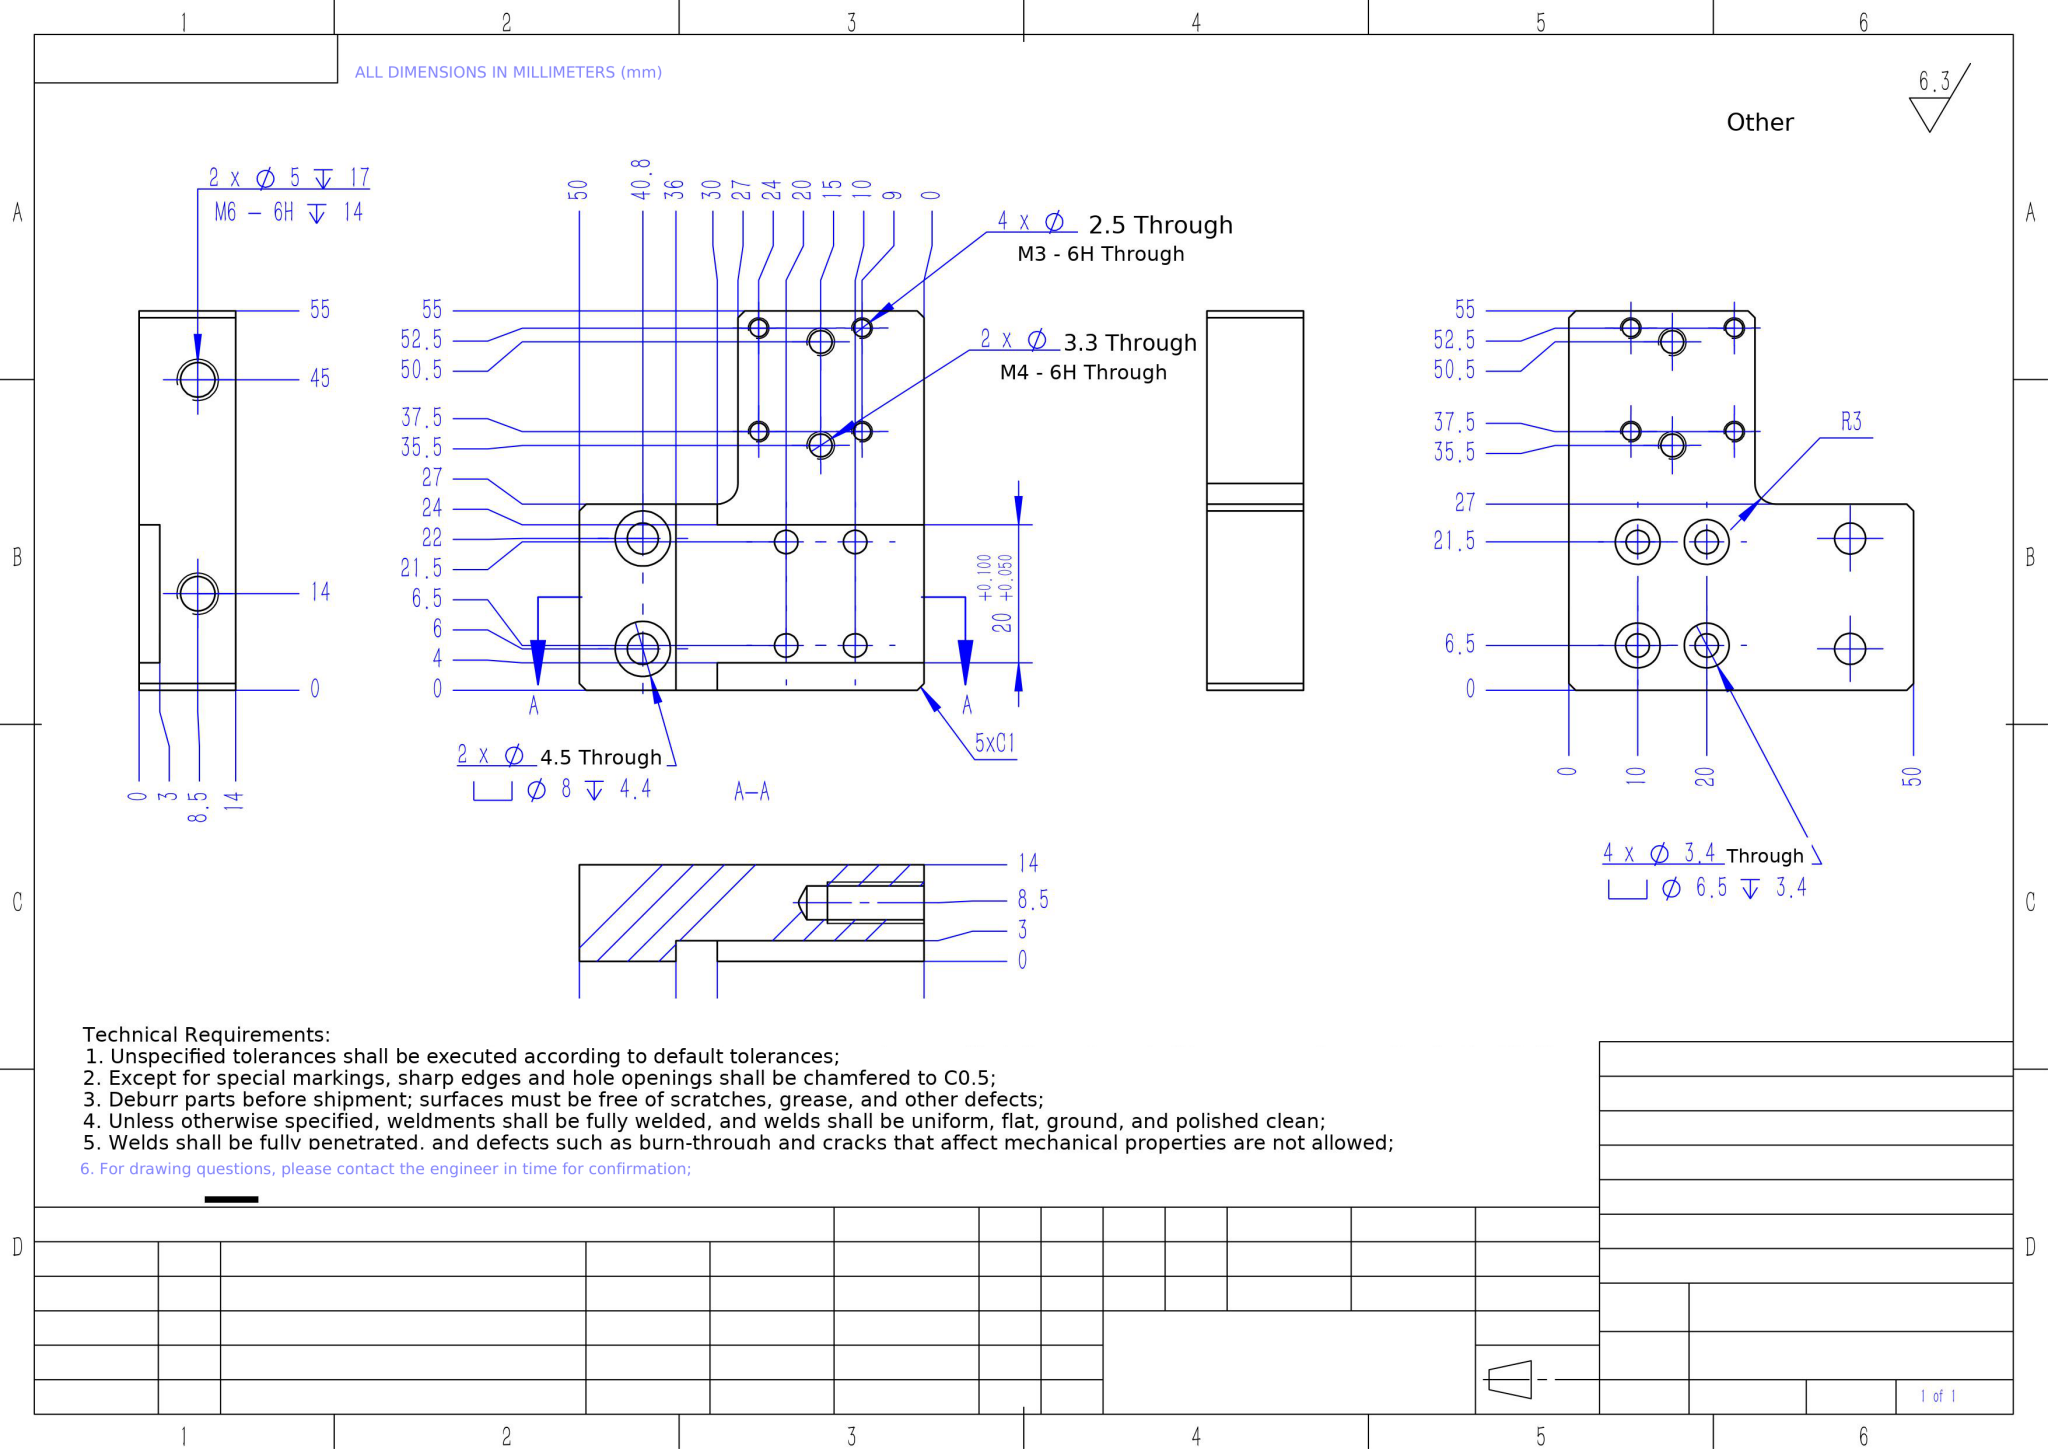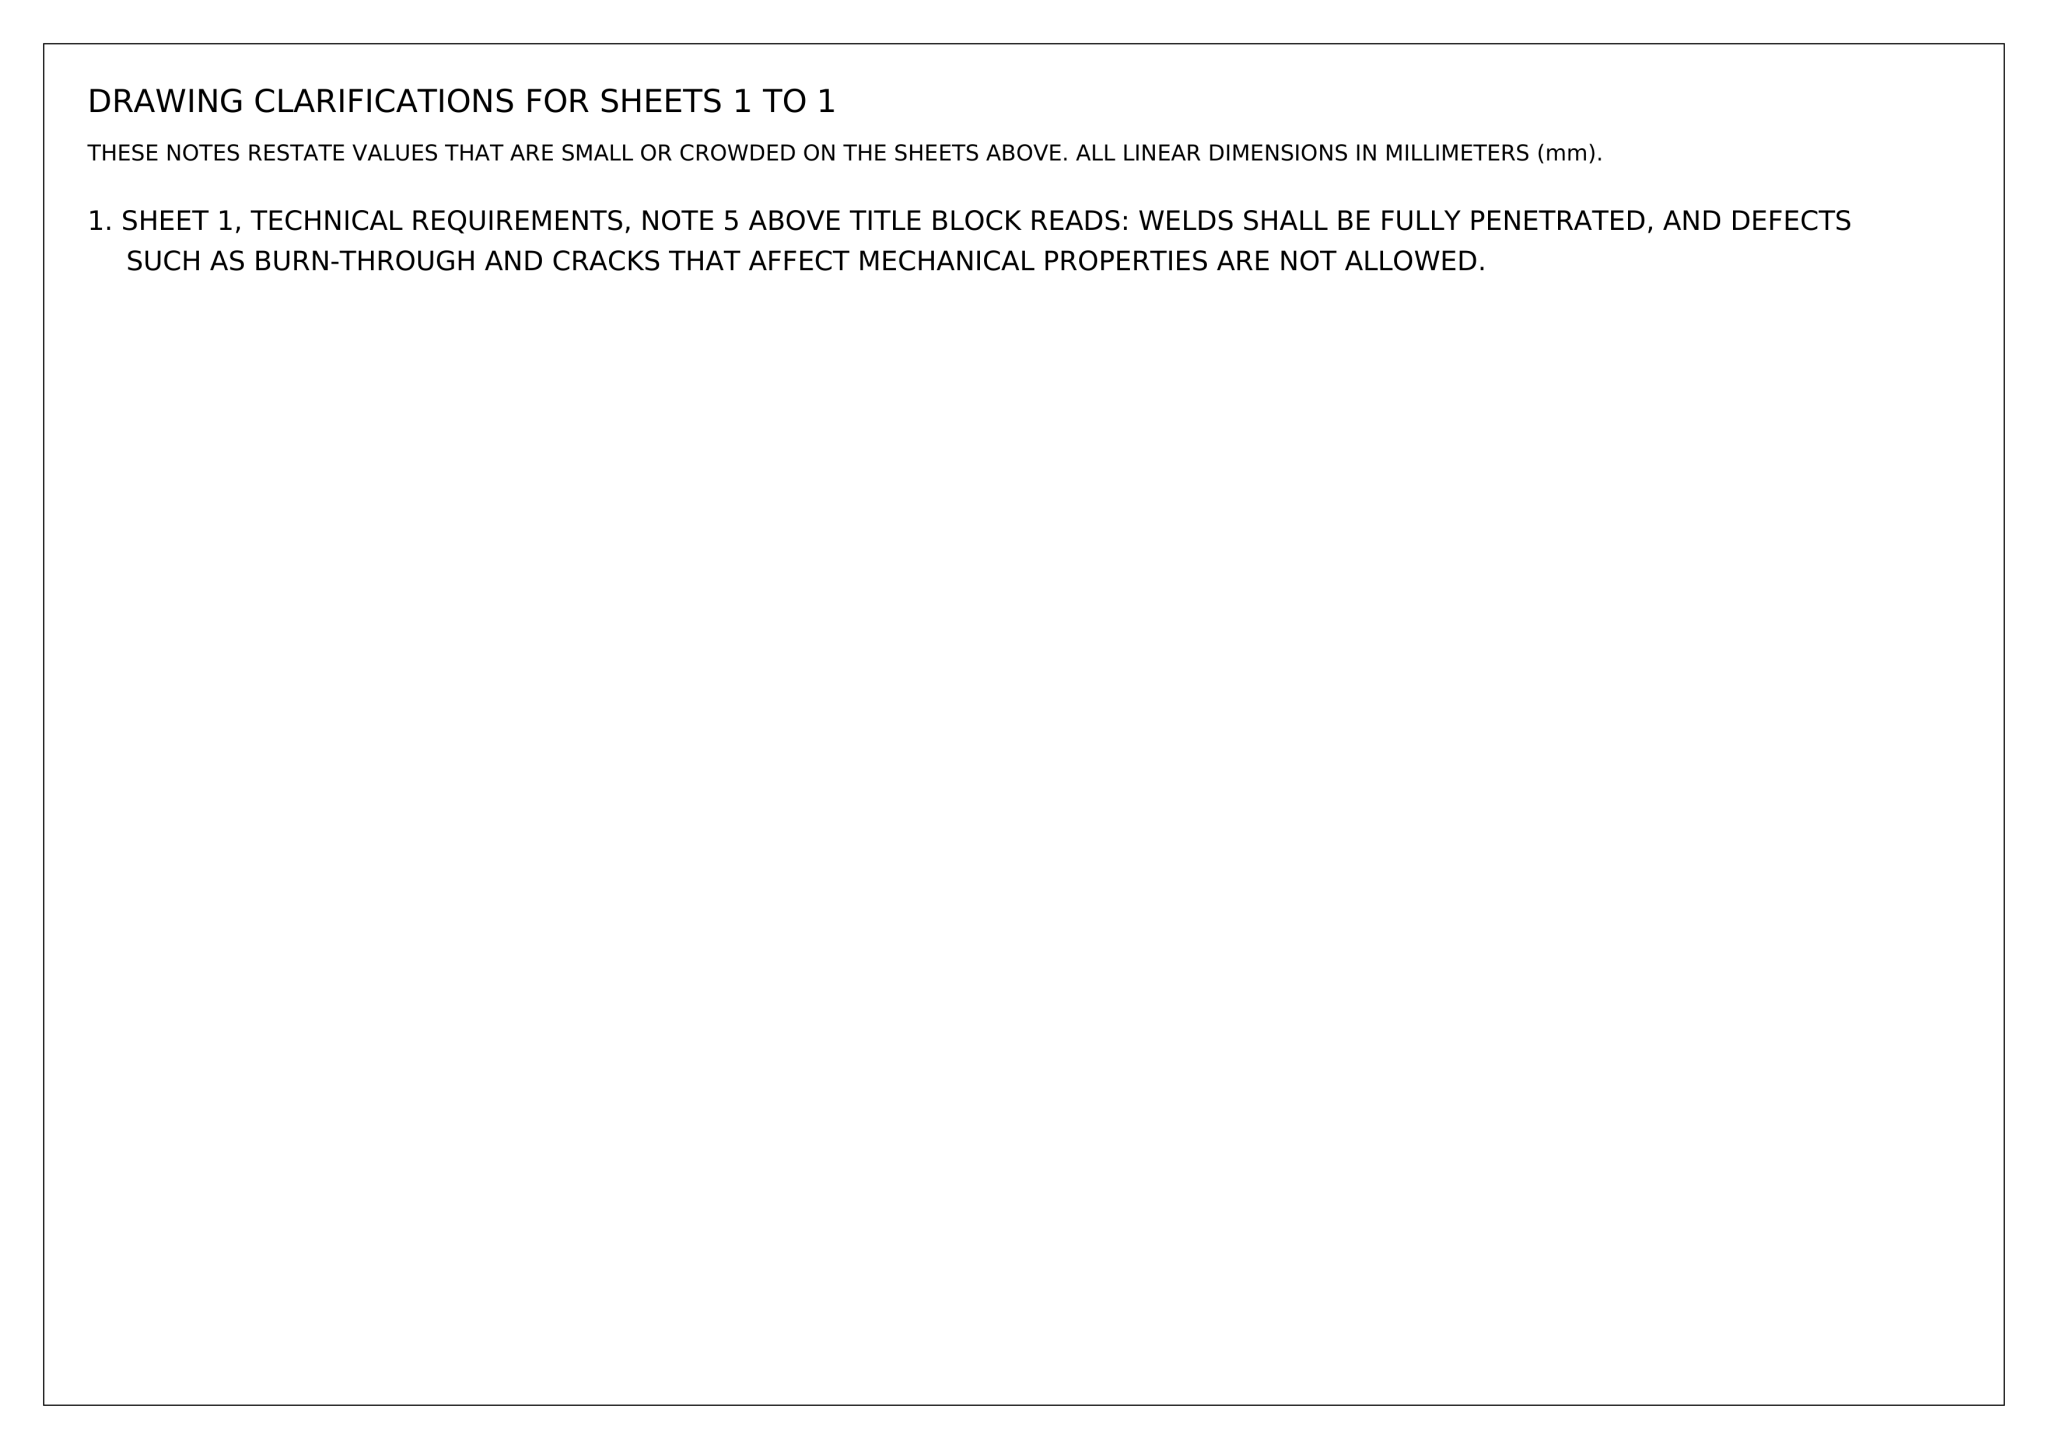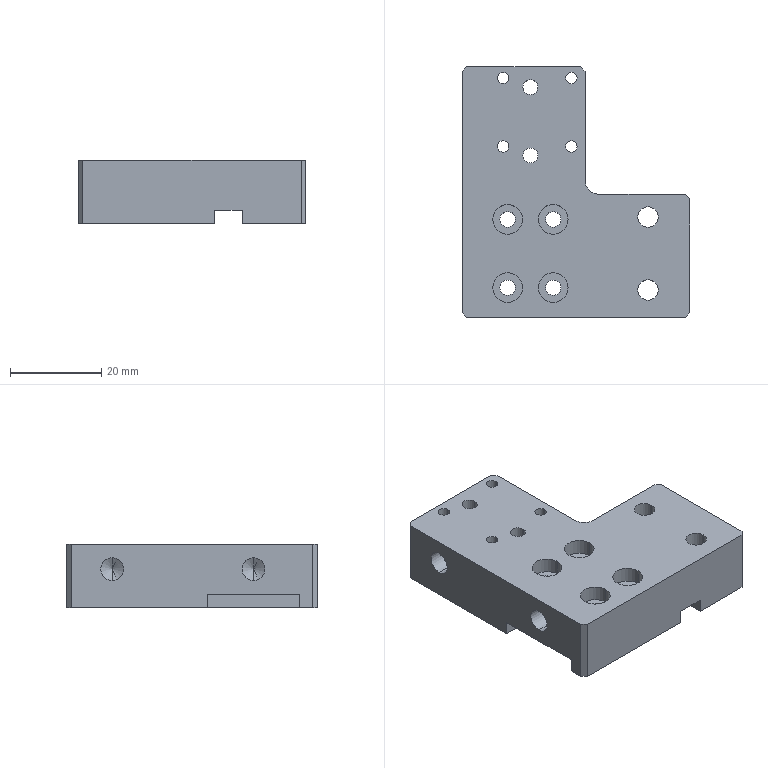Part | NX | mm | 1 solid | 72 faces | box 50 x 55 x 14 mm | volume 24513 mm3 | cylinder 41 | plane 27 | cone 4 | commonest cylinder face diameters 2.5 x8 6.5 x8 3.4 x8 3.3 x4 5 x4 8 x4 4.5 x4 6 x1